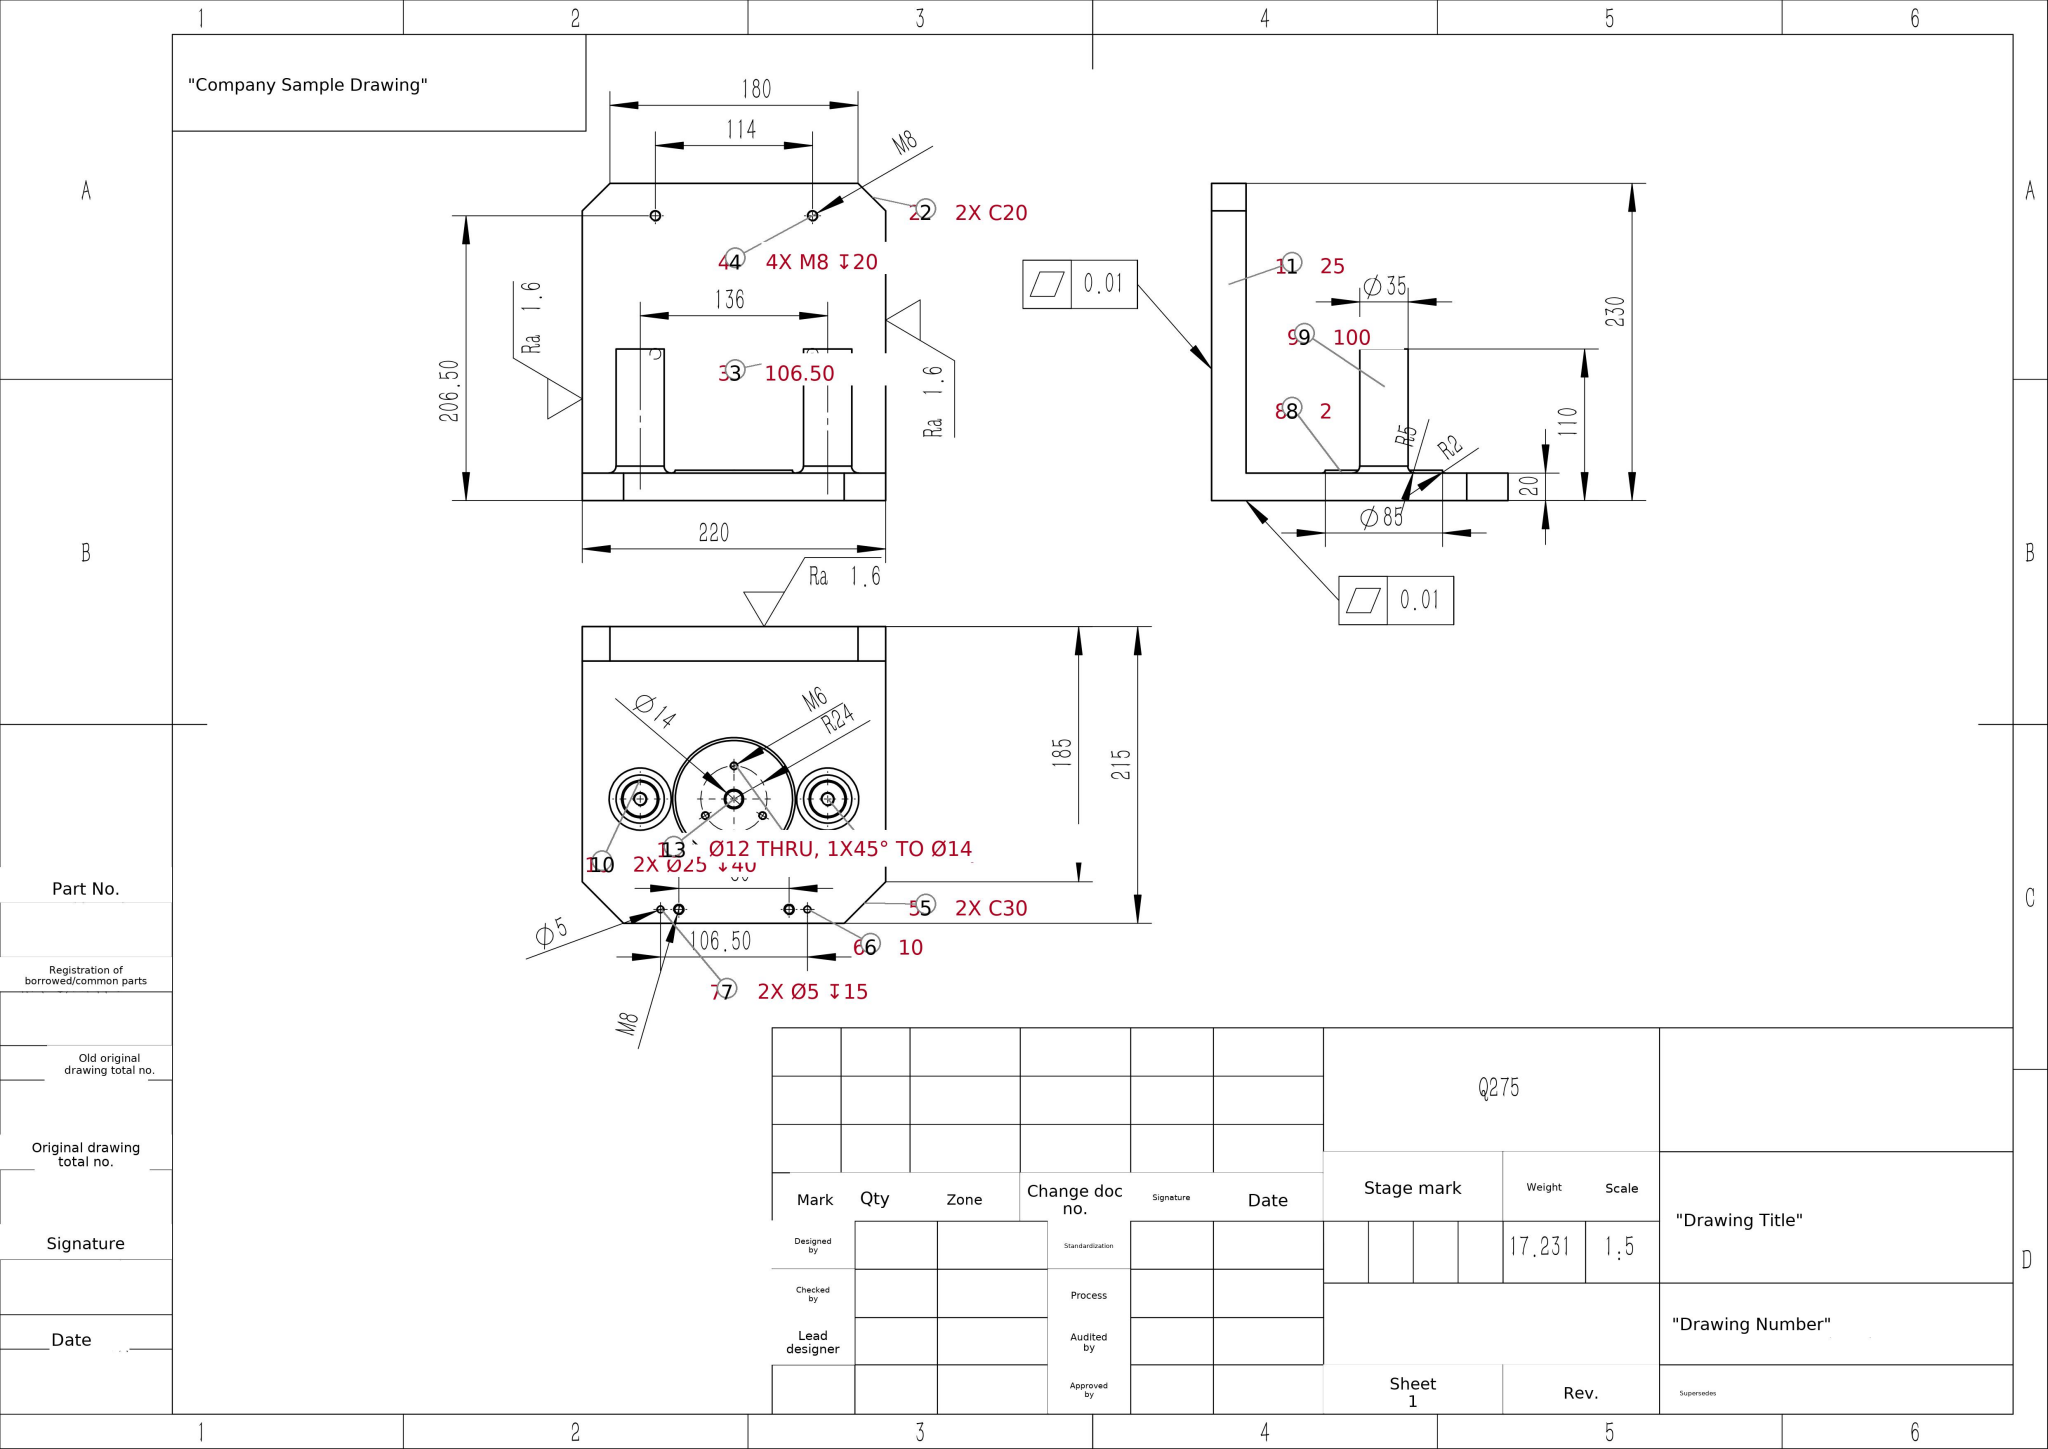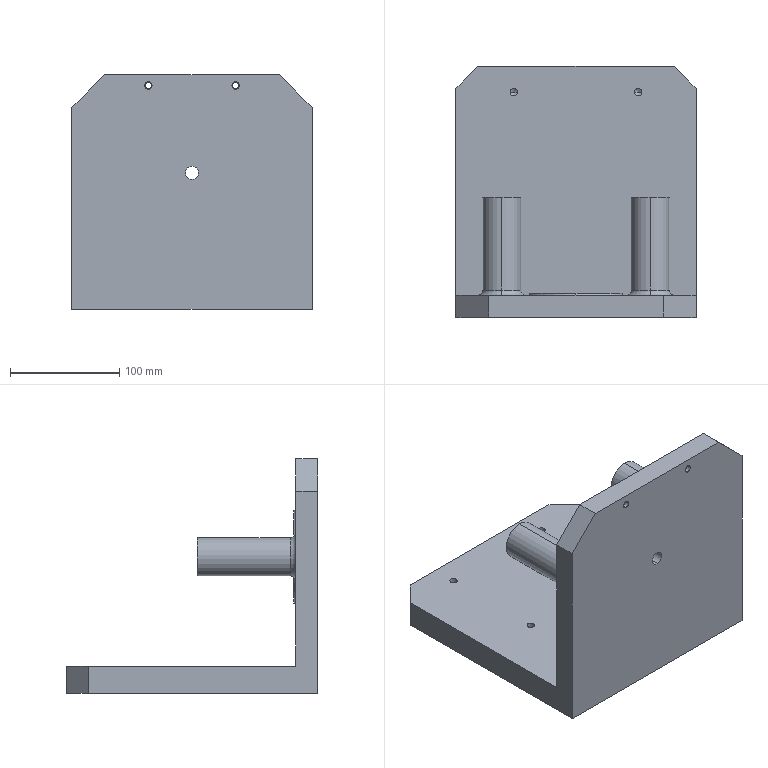Part | SolidWorks | mm | material Q275 | 1 solid | 89 faces | box 220 x 230 x 215 mm | volume 2209129 mm3 | cylinder 36 | cone 28 | plane 19 | torus 6 | commonest cylinder face diameters 6.8 x12 5 x10 8.5 x4 25 x4 35 x4 12 x2